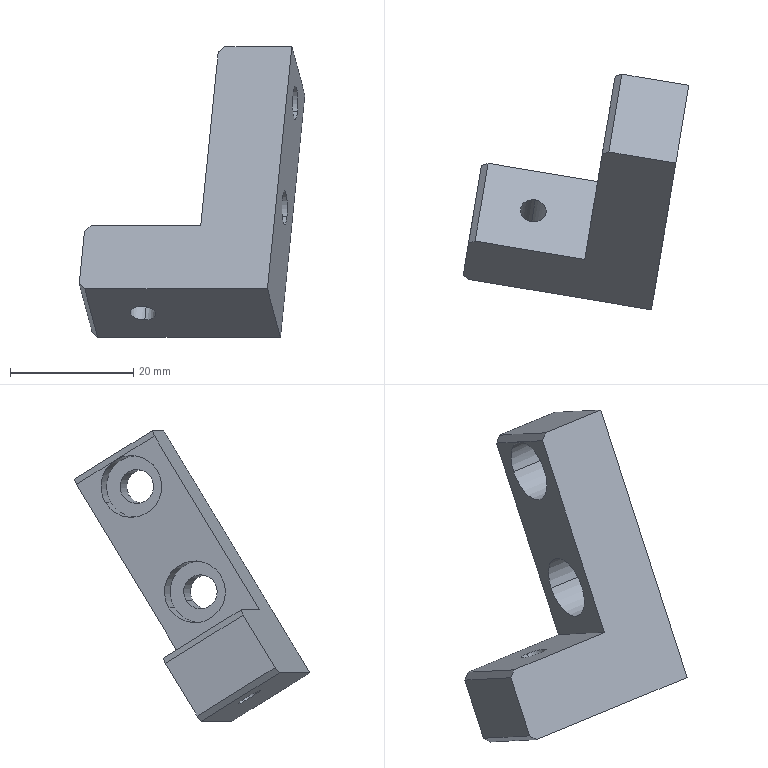Component | SolidWorks | 14AC-24-1-010-1 | 1 solid | 23 faces | box 36.54 x 38.12 x 47.06 mm | volume 10349 mm3 | plane 13 | cylinder 10 | commonest cylinder face diameters 10 x4 5.5 x4 4.2 x2
STEP:
#1=COLOUR_RGB('',0.7922,0.8196,0.9333);
#2=FILL_AREA_STYLE_COLOUR('',#1);
#3=FILL_AREA_STYLE('',(#2));
#4=SURFACE_STYLE_FILL_AREA(#3);
#5=SURFACE_SIDE_STYLE('',(#4));
#6=SURFACE_STYLE_USAGE(.BOTH.,#5);
#7=PRESENTATION_STYLE_ASSIGNMENT((#6));
#8=CARTESIAN_POINT('',(13.586,-5.303,-6.958));
#9=VERTEX_POINT('',#8);
#10=CARTESIAN_POINT('',(13.531,-5.634,-6.753));
#11=VERTEX_POINT('',#10);
#12=CARTESIAN_POINT('',(13.559,-5.468,-6.856));
#13=DIRECTION('',(-0.9864,0.1642,0.));
#14=DIRECTION('',(-0.1401,-0.8413,0.5222));
#15=AXIS2_PLACEMENT_3D('',#12,#13,#14);
#16=CIRCLE('',#15,0.1969);
#17=EDGE_CURVE('',#9,#11,#16,.T.);
#18=ORIENTED_EDGE('',*,*,#17,.F.);
#19=CARTESIAN_POINT('',(13.377,-5.268,-6.958));
#20=VERTEX_POINT('',#19);
#21=CARTESIAN_POINT('',(13.377,-5.268,-6.958));
#22=DIRECTION('',(-0.9864,0.1642,0.));
#23=VECTOR('',#22,39.37);
#24=LINE('',#21,#23);
#25=EDGE_CURVE('',#9,#20,#24,.T.);
#26=ORIENTED_EDGE('',*,*,#25,.T.);
#27=CARTESIAN_POINT('',(13.321,-5.599,-6.753));
#28=VERTEX_POINT('',#27);
#29=CARTESIAN_POINT('',(13.349,-5.433,-6.856));
#30=DIRECTION('',(-0.9864,0.1642,0.));
#31=DIRECTION('',(-0.1401,-0.8413,0.5222));
#32=AXIS2_PLACEMENT_3D('',#29,#30,#31);
#33=CIRCLE('',#32,0.1969);
#34=EDGE_CURVE('',#20,#28,#33,.T.);
#35=ORIENTED_EDGE('',*,*,#34,.T.);
#36=CARTESIAN_POINT('',(13.321,-5.599,-6.753));
#37=DIRECTION('',(-0.9864,0.1642,0.));
#38=VECTOR('',#37,39.37);
#39=LINE('',#36,#38);
#40=EDGE_CURVE('',#11,#28,#39,.T.);
#41=ORIENTED_EDGE('',*,*,#40,.F.);
#42=EDGE_LOOP('',(#18,#26,#35,#41));
#43=FACE_OUTER_BOUND('',#42,.T.);
#44=CARTESIAN_POINT('',(13.349,-5.433,-6.856));
#45=DIRECTION('',(-0.9864,0.1642,0.));
#46=DIRECTION('',(-0.1401,-0.8413,0.5222));
#47=AXIS2_PLACEMENT_3D('',#44,#45,#46);
#48=CYLINDRICAL_SURFACE('',#47,0.1969);
#49=ADVANCED_FACE('',(#43),#48,.F.);
#50=CARTESIAN_POINT('',(13.83,-5.42,-6.912));
#51=VERTEX_POINT('',#50);
#52=CARTESIAN_POINT('',(13.8,-5.602,-6.799));
#53=VERTEX_POINT('',#52);
#54=CARTESIAN_POINT('',(13.815,-5.511,-6.856));
#55=DIRECTION('',(-0.9864,0.1642,0.));
#56=DIRECTION('',(-0.1401,-0.8413,0.5222));
#57=AXIS2_PLACEMENT_3D('',#54,#55,#56);
#58=CIRCLE('',#57,0.1083);
#59=EDGE_CURVE('',#51,#53,#58,.T.);
#60=ORIENTED_EDGE('',*,*,#59,.F.);
#61=CARTESIAN_POINT('',(13.574,-5.377,-6.912));
#62=VERTEX_POINT('',#61);
#63=CARTESIAN_POINT('',(13.364,-5.342,-6.912));
#64=DIRECTION('',(-0.9864,0.1642,0.));
#65=VECTOR('',#64,39.37);
#66=LINE('',#63,#65);
#67=EDGE_CURVE('',#51,#62,#66,.T.);
#68=ORIENTED_EDGE('',*,*,#67,.T.);
#69=CARTESIAN_POINT('',(13.544,-5.559,-6.799));
#70=VERTEX_POINT('',#69);
#71=CARTESIAN_POINT('',(13.559,-5.468,-6.856));
#72=DIRECTION('',(-0.9864,0.1642,0.));
#73=DIRECTION('',(-0.1401,-0.8413,0.5222));
#74=AXIS2_PLACEMENT_3D('',#71,#72,#73);
#75=CIRCLE('',#74,0.1083);
#76=EDGE_CURVE('',#62,#70,#75,.T.);
#77=ORIENTED_EDGE('',*,*,#76,.T.);
#78=CARTESIAN_POINT('',(13.334,-5.525,-6.799));
#79=DIRECTION('',(-0.9864,0.1642,0.));
#80=VECTOR('',#79,39.37);
#81=LINE('',#78,#80);
#82=EDGE_CURVE('',#53,#70,#81,.T.);
#83=ORIENTED_EDGE('',*,*,#82,.F.);
#84=EDGE_LOOP('',(#60,#68,#77,#83));
#85=FACE_OUTER_BOUND('',#84,.T.);
#86=CARTESIAN_POINT('',(13.349,-5.433,-6.856));
#87=DIRECTION('',(-0.9864,0.1642,0.));
#88=DIRECTION('',(-0.1401,-0.8413,0.5222));
#89=AXIS2_PLACEMENT_3D('',#86,#87,#88);
#90=CYLINDRICAL_SURFACE('',#89,0.1083);
#91=ADVANCED_FACE('',(#85),#90,.F.);
#92=CARTESIAN_POINT('',(13.654,-4.897,-6.287));
#93=VERTEX_POINT('',#92);
#94=CARTESIAN_POINT('',(13.599,-5.228,-6.081));
#95=VERTEX_POINT('',#94);
#96=CARTESIAN_POINT('',(13.626,-5.063,-6.184));
#97=DIRECTION('',(-0.9864,0.1642,0.));
#98=DIRECTION('',(-0.1401,-0.8413,0.5222));
#99=AXIS2_PLACEMENT_3D('',#96,#97,#98);
#100=CIRCLE('',#99,0.1969);
#101=EDGE_CURVE('',#93,#95,#100,.T.);
#102=ORIENTED_EDGE('',*,*,#101,.F.);
#103=CARTESIAN_POINT('',(13.444,-4.862,-6.287));
#104=VERTEX_POINT('',#103);
#105=CARTESIAN_POINT('',(13.444,-4.862,-6.287));
#106=DIRECTION('',(-0.9864,0.1642,0.));
#107=VECTOR('',#106,39.37);
#108=LINE('',#105,#107);
#109=EDGE_CURVE('',#93,#104,#108,.T.);
#110=ORIENTED_EDGE('',*,*,#109,.T.);
#111=CARTESIAN_POINT('',(13.389,-5.194,-6.081));
#112=VERTEX_POINT('',#111);
#113=CARTESIAN_POINT('',(13.417,-5.028,-6.184));
#114=DIRECTION('',(-0.9864,0.1642,0.));
#115=DIRECTION('',(-0.1401,-0.8413,0.5222));
#116=AXIS2_PLACEMENT_3D('',#113,#114,#115);
#117=CIRCLE('',#116,0.1969);
#118=EDGE_CURVE('',#104,#112,#117,.T.);
#119=ORIENTED_EDGE('',*,*,#118,.T.);
#120=CARTESIAN_POINT('',(13.389,-5.194,-6.081));
#121=DIRECTION('',(-0.9864,0.1642,0.));
#122=VECTOR('',#121,39.37);
#123=LINE('',#120,#122);
#124=EDGE_CURVE('',#95,#112,#123,.T.);
#125=ORIENTED_EDGE('',*,*,#124,.F.);
#126=EDGE_LOOP('',(#102,#110,#119,#125));
#127=FACE_OUTER_BOUND('',#126,.T.);
#128=CARTESIAN_POINT('',(13.417,-5.028,-6.184));
#129=DIRECTION('',(-0.9864,0.1642,0.));
#130=DIRECTION('',(-0.1401,-0.8413,0.5222));
#131=AXIS2_PLACEMENT_3D('',#128,#129,#130);
#132=CYLINDRICAL_SURFACE('',#131,0.1969);
#133=ADVANCED_FACE('',(#127),#132,.F.);
#134=CARTESIAN_POINT('',(13.898,-5.014,-6.241));
#135=VERTEX_POINT('',#134);
#136=CARTESIAN_POINT('',(13.867,-5.197,-6.127));
#137=VERTEX_POINT('',#136);
#138=CARTESIAN_POINT('',(13.883,-5.106,-6.184));
#139=DIRECTION('',(-0.9864,0.1642,0.));
#140=DIRECTION('',(-0.1401,-0.8413,0.5222));
#141=AXIS2_PLACEMENT_3D('',#138,#139,#140);
#142=CIRCLE('',#141,0.1083);
#143=EDGE_CURVE('',#135,#137,#142,.T.);
#144=ORIENTED_EDGE('',*,*,#143,.F.);
#145=CARTESIAN_POINT('',(13.641,-4.972,-6.241));
#146=VERTEX_POINT('',#145);
#147=CARTESIAN_POINT('',(13.432,-4.937,-6.241));
#148=DIRECTION('',(-0.9864,0.1642,0.));
#149=VECTOR('',#148,39.37);
#150=LINE('',#147,#149);
#151=EDGE_CURVE('',#135,#146,#150,.T.);
#152=ORIENTED_EDGE('',*,*,#151,.T.);
#153=CARTESIAN_POINT('',(13.611,-5.154,-6.127));
#154=VERTEX_POINT('',#153);
#155=CARTESIAN_POINT('',(13.626,-5.063,-6.184));
#156=DIRECTION('',(-0.9864,0.1642,0.));
#157=DIRECTION('',(-0.1401,-0.8413,0.5222));
#158=AXIS2_PLACEMENT_3D('',#155,#156,#157);
#159=CIRCLE('',#158,0.1083);
#160=EDGE_CURVE('',#146,#154,#159,.T.);
#161=ORIENTED_EDGE('',*,*,#160,.T.);
#162=CARTESIAN_POINT('',(13.401,-5.119,-6.127));
#163=DIRECTION('',(-0.9864,0.1642,0.));
#164=VECTOR('',#163,39.37);
#165=LINE('',#162,#164);
#166=EDGE_CURVE('',#137,#154,#165,.T.);
#167=ORIENTED_EDGE('',*,*,#166,.F.);
#168=EDGE_LOOP('',(#144,#152,#161,#167));
#169=FACE_OUTER_BOUND('',#168,.T.);
#170=CARTESIAN_POINT('',(13.417,-5.028,-6.184));
#171=DIRECTION('',(-0.9864,0.1642,0.));
#172=DIRECTION('',(-0.1401,-0.8413,0.5222));
#173=AXIS2_PLACEMENT_3D('',#170,#171,#172);
#174=CYLINDRICAL_SURFACE('',#173,0.1083);
#175=ADVANCED_FACE('',(#169),#174,.F.);
#176=CARTESIAN_POINT('',(12.924,-5.708,-7.57));
#177=VERTEX_POINT('',#176);
#178=CARTESIAN_POINT('',(12.901,-5.847,-7.484));
#179=VERTEX_POINT('',#178);
#180=CARTESIAN_POINT('',(12.913,-5.778,-7.527));
#181=DIRECTION('',(0.08576,0.5151,0.8529));
#182=DIRECTION('',(0.9864,-0.1642,0.));
#183=AXIS2_PLACEMENT_3D('',#180,#181,#182);
#184=CIRCLE('',#183,0.08268);
#185=EDGE_CURVE('',#177,#179,#184,.T.);
#186=ORIENTED_EDGE('',*,*,#185,.F.);
#187=CARTESIAN_POINT('',(12.965,-5.465,-7.167));
#188=VERTEX_POINT('',#187);
#189=CARTESIAN_POINT('',(12.965,-5.465,-7.167));
#190=DIRECTION('',(0.08576,0.5151,0.8529));
#191=VECTOR('',#190,39.37);
#192=LINE('',#189,#191);
#193=EDGE_CURVE('',#177,#188,#192,.T.);
#194=ORIENTED_EDGE('',*,*,#193,.T.);
#195=CARTESIAN_POINT('',(12.941,-5.604,-7.081));
#196=VERTEX_POINT('',#195);
#197=CARTESIAN_POINT('',(12.953,-5.534,-7.124));
#198=DIRECTION('',(0.08576,0.5151,0.8529));
#199=DIRECTION('',(-0.1401,-0.8413,0.5222));
#200=AXIS2_PLACEMENT_3D('',#197,#198,#199);
#201=CIRCLE('',#200,0.08268);
#202=EDGE_CURVE('',#188,#196,#201,.T.);
#203=ORIENTED_EDGE('',*,*,#202,.T.);
#204=CARTESIAN_POINT('',(12.941,-5.604,-7.081));
#205=DIRECTION('',(0.08576,0.5151,0.8529));
#206=VECTOR('',#205,39.37);
#207=LINE('',#204,#206);
#208=EDGE_CURVE('',#179,#196,#207,.T.);
#209=ORIENTED_EDGE('',*,*,#208,.F.);
#210=EDGE_LOOP('',(#186,#194,#203,#209));
#211=FACE_OUTER_BOUND('',#210,.T.);
#212=CARTESIAN_POINT('',(12.953,-5.534,-7.124));
#213=DIRECTION('',(0.08576,0.5151,0.8529));
#214=DIRECTION('',(-0.1401,-0.8413,0.5222));
#215=AXIS2_PLACEMENT_3D('',#212,#213,#214);
#216=CYLINDRICAL_SURFACE('',#215,0.08268);
#217=ADVANCED_FACE('',(#211),#216,.F.);
#218=CARTESIAN_POINT('',(13.517,-4.664,-6.137));
#219=VERTEX_POINT('',#218);
#220=CARTESIAN_POINT('',(13.944,-4.735,-6.137));
#221=VERTEX_POINT('',#220);
#222=CARTESIAN_POINT('',(13.944,-4.735,-6.137));
#223=DIRECTION('',(0.9864,-0.1642,-0.));
#224=VECTOR('',#223,39.37);
#225=LINE('',#222,#224);
#226=EDGE_CURVE('',#219,#221,#225,.T.);
#227=ORIENTED_EDGE('',*,*,#226,.F.);
#228=CARTESIAN_POINT('',(13.434,-5.161,-5.828));
#229=VERTEX_POINT('',#228);
#230=CARTESIAN_POINT('',(13.517,-4.664,-6.137));
#231=DIRECTION('',(-0.1401,-0.8413,0.5222));
#232=VECTOR('',#231,39.37);
#233=LINE('',#230,#232);
#234=EDGE_CURVE('',#219,#229,#233,.T.);
#235=ORIENTED_EDGE('',*,*,#234,.T.);
#236=CARTESIAN_POINT('',(13.861,-5.232,-5.828));
#237=VERTEX_POINT('',#236);
#238=CARTESIAN_POINT('',(13.861,-5.232,-5.828));
#239=DIRECTION('',(0.9864,-0.1642,-0.));
#240=VECTOR('',#239,39.37);
#241=LINE('',#238,#240);
#242=EDGE_CURVE('',#229,#237,#241,.T.);
#243=ORIENTED_EDGE('',*,*,#242,.T.);
#244=CARTESIAN_POINT('',(13.944,-4.735,-6.137));
#245=DIRECTION('',(-0.1401,-0.8413,0.5222));
#246=VECTOR('',#245,39.37);
#247=LINE('',#244,#246);
#248=EDGE_CURVE('',#221,#237,#247,.T.);
#249=ORIENTED_EDGE('',*,*,#248,.F.);
#250=EDGE_LOOP('',(#227,#235,#243,#249));
#251=FACE_OUTER_BOUND('',#250,.T.);
#252=CARTESIAN_POINT('',(13.944,-4.735,-6.137));
#253=DIRECTION('',(-0.08576,-0.5151,-0.8529));
#254=DIRECTION('',(-0.9864,0.1642,0.));
#255=AXIS2_PLACEMENT_3D('',#252,#253,#254);
#256=PLANE('',#255);
#257=ADVANCED_FACE('',(#251),#256,.F.);
#258=CARTESIAN_POINT('',(13.815,-5.511,-6.856));
#259=DIRECTION('',(-0.9864,0.1642,0.));
#260=DIRECTION('',(-0.1401,-0.8413,0.5222));
#261=AXIS2_PLACEMENT_3D('',#258,#259,#260);
#262=CIRCLE('',#261,0.1083);
#263=EDGE_CURVE('',#53,#51,#262,.T.);
#264=ORIENTED_EDGE('',*,*,#263,.T.);
#265=ORIENTED_EDGE('',*,*,#59,.T.);
#266=EDGE_LOOP('',(#264,#265));
#267=FACE_BOUND('',#266,.T.);
#268=CARTESIAN_POINT('',(13.883,-5.106,-6.184));
#269=DIRECTION('',(-0.9864,0.1642,0.));
#270=DIRECTION('',(-0.1401,-0.8413,0.5222));
#271=AXIS2_PLACEMENT_3D('',#268,#269,#270);
#272=CIRCLE('',#271,0.1083);
#273=EDGE_CURVE('',#137,#135,#272,.T.);
#274=ORIENTED_EDGE('',*,*,#273,.T.);
#275=ORIENTED_EDGE('',*,*,#143,.T.);
#276=EDGE_LOOP('',(#274,#275));
#277=FACE_BOUND('',#276,.T.);
#278=CARTESIAN_POINT('',(13.706,-6.165,-7.373));
#279=VERTEX_POINT('',#278);
#280=CARTESIAN_POINT('',(13.706,-6.165,-7.373));
#281=DIRECTION('',(-0.08576,-0.5151,-0.8529));
#282=VECTOR('',#281,39.37);
#283=LINE('',#280,#282);
#284=EDGE_CURVE('',#237,#279,#283,.T.);
#285=ORIENTED_EDGE('',*,*,#284,.T.);
#286=CARTESIAN_POINT('',(13.789,-5.668,-7.681));
#287=VERTEX_POINT('',#286);
#288=CARTESIAN_POINT('',(13.789,-5.668,-7.681));
#289=DIRECTION('',(-0.1401,-0.8413,0.5222));
#290=VECTOR('',#289,39.37);
#291=LINE('',#288,#290);
#292=EDGE_CURVE('',#287,#279,#291,.T.);
#293=ORIENTED_EDGE('',*,*,#292,.F.);
#294=CARTESIAN_POINT('',(13.789,-5.668,-7.681));
#295=DIRECTION('',(-0.08576,-0.5151,-0.8529));
#296=VECTOR('',#295,39.37);
#297=LINE('',#294,#296);
#298=EDGE_CURVE('',#221,#287,#297,.T.);
#299=ORIENTED_EDGE('',*,*,#298,.F.);
#300=ORIENTED_EDGE('',*,*,#248,.T.);
#301=EDGE_LOOP('',(#285,#293,#299,#300));
#302=FACE_OUTER_BOUND('',#301,.T.);
#303=CARTESIAN_POINT('',(13.789,-5.668,-7.681));
#304=DIRECTION('',(-0.9864,0.1642,0.));
#305=DIRECTION('',(-0.1401,-0.8413,0.5222));
#306=AXIS2_PLACEMENT_3D('',#303,#304,#305);
#307=PLANE('',#306);
#308=ADVANCED_FACE('',(#267,#277,#302),#307,.F.);
#309=CARTESIAN_POINT('',(12.913,-5.778,-7.527));
#310=DIRECTION('',(0.08576,0.5151,0.8529));
#311=DIRECTION('',(0.9864,-0.1642,0.));
#312=AXIS2_PLACEMENT_3D('',#309,#310,#311);
#313=CIRCLE('',#312,0.08268);
#314=EDGE_CURVE('',#179,#177,#313,.T.);
#315=ORIENTED_EDGE('',*,*,#314,.T.);
#316=ORIENTED_EDGE('',*,*,#185,.T.);
#317=EDGE_LOOP('',(#315,#316));
#318=FACE_BOUND('',#317,.T.);
#319=CARTESIAN_POINT('',(12.541,-5.971,-7.373));
#320=VERTEX_POINT('',#319);
#321=CARTESIAN_POINT('',(13.706,-6.165,-7.373));
#322=DIRECTION('',(-0.9864,0.1642,0.));
#323=VECTOR('',#322,39.37);
#324=LINE('',#321,#323);
#325=EDGE_CURVE('',#279,#320,#324,.T.);
#326=ORIENTED_EDGE('',*,*,#325,.T.);
#327=CARTESIAN_POINT('',(12.624,-5.474,-7.681));
#328=VERTEX_POINT('',#327);
#329=CARTESIAN_POINT('',(12.624,-5.474,-7.681));
#330=DIRECTION('',(0.1401,0.8413,-0.5222));
#331=VECTOR('',#330,39.37);
#332=LINE('',#329,#331);
#333=EDGE_CURVE('',#320,#328,#332,.T.);
#334=ORIENTED_EDGE('',*,*,#333,.T.);
#335=CARTESIAN_POINT('',(13.789,-5.668,-7.681));
#336=DIRECTION('',(-0.9864,0.1642,0.));
#337=VECTOR('',#336,39.37);
#338=LINE('',#335,#337);
#339=EDGE_CURVE('',#287,#328,#338,.T.);
#340=ORIENTED_EDGE('',*,*,#339,.F.);
#341=ORIENTED_EDGE('',*,*,#292,.T.);
#342=EDGE_LOOP('',(#326,#334,#340,#341));
#343=FACE_OUTER_BOUND('',#342,.T.);
#344=CARTESIAN_POINT('',(13.789,-5.668,-7.681));
#345=DIRECTION('',(0.08576,0.5151,0.8529));
#346=DIRECTION('',(0.9864,-0.1642,-0.));
#347=AXIS2_PLACEMENT_3D('',#344,#345,#346);
#348=PLANE('',#347);
#349=ADVANCED_FACE('',(#318,#343),#348,.F.);
#350=CARTESIAN_POINT('',(12.588,-5.447,-7.648));
#351=VERTEX_POINT('',#350);
#352=CARTESIAN_POINT('',(12.622,-5.245,-7.312));
#353=VERTEX_POINT('',#352);
#354=CARTESIAN_POINT('',(12.585,-5.468,-7.681));
#355=DIRECTION('',(0.08576,0.5151,0.8529));
#356=VECTOR('',#355,39.37);
#357=LINE('',#354,#356);
#358=EDGE_CURVE('',#351,#353,#357,.T.);
#359=ORIENTED_EDGE('',*,*,#358,.F.);
#360=CARTESIAN_POINT('',(12.506,-5.944,-7.339));
#361=VERTEX_POINT('',#360);
#362=CARTESIAN_POINT('',(12.588,-5.447,-7.648));
#363=DIRECTION('',(-0.1401,-0.8413,0.5222));
#364=VECTOR('',#363,39.37);
#365=LINE('',#362,#364);
#366=EDGE_CURVE('',#351,#361,#365,.T.);
#367=ORIENTED_EDGE('',*,*,#366,.T.);
#368=CARTESIAN_POINT('',(12.539,-5.742,-7.004));
#369=VERTEX_POINT('',#368);
#370=CARTESIAN_POINT('',(12.502,-5.965,-7.373));
#371=DIRECTION('',(0.08576,0.5151,0.8529));
#372=VECTOR('',#371,39.37);
#373=LINE('',#370,#372);
#374=EDGE_CURVE('',#361,#369,#373,.T.);
#375=ORIENTED_EDGE('',*,*,#374,.T.);
#376=CARTESIAN_POINT('',(12.622,-5.245,-7.312));
#377=DIRECTION('',(0.1401,0.8413,-0.5222));
#378=VECTOR('',#377,39.37);
#379=LINE('',#376,#378);
#380=EDGE_CURVE('',#369,#353,#379,.T.);
#381=ORIENTED_EDGE('',*,*,#380,.T.);
#382=EDGE_LOOP('',(#359,#367,#375,#381));
#383=FACE_OUTER_BOUND('',#382,.T.);
#384=CARTESIAN_POINT('',(12.585,-5.468,-7.681));
#385=DIRECTION('',(0.9864,-0.1642,-0.));
#386=DIRECTION('',(0.1401,0.8413,-0.5222));
#387=AXIS2_PLACEMENT_3D('',#384,#385,#386);
#388=PLANE('',#387);
#389=ADVANCED_FACE('',(#383),#388,.F.);
#390=ORIENTED_EDGE('',*,*,#339,.T.);
#391=CARTESIAN_POINT('',(12.473,-5.361,-7.539));
#392=DIRECTION('',(-0.6369,0.4803,0.6031));
#393=VECTOR('',#392,39.37);
#394=LINE('',#391,#393);
#395=EDGE_CURVE('',#328,#351,#394,.T.);
#396=ORIENTED_EDGE('',*,*,#395,.T.);
#397=ORIENTED_EDGE('',*,*,#358,.T.);
#398=CARTESIAN_POINT('',(12.664,-5.231,-7.278));
#399=VERTEX_POINT('',#398);
#400=CARTESIAN_POINT('',(13.203,-5.055,-6.85));
#401=DIRECTION('',(0.7581,0.2481,0.6031));
#402=VECTOR('',#401,39.37);
#403=LINE('',#400,#402);
#404=EDGE_CURVE('',#353,#399,#403,.T.);
#405=ORIENTED_EDGE('',*,*,#404,.T.);
#406=CARTESIAN_POINT('',(13.363,-5.347,-7.278));
#407=VERTEX_POINT('',#406);
#408=CARTESIAN_POINT('',(13.363,-5.347,-7.278));
#409=DIRECTION('',(-0.9864,0.1642,0.));
#410=VECTOR('',#409,39.37);
#411=LINE('',#408,#410);
#412=EDGE_CURVE('',#407,#399,#411,.T.);
#413=ORIENTED_EDGE('',*,*,#412,.F.);
#414=CARTESIAN_POINT('',(13.475,-4.678,-6.17));
#415=VERTEX_POINT('',#414);
#416=CARTESIAN_POINT('',(13.478,-4.658,-6.137));
#417=DIRECTION('',(-0.08576,-0.5151,-0.8529));
#418=VECTOR('',#417,39.37);
#419=LINE('',#416,#418);
#420=EDGE_CURVE('',#415,#407,#419,.T.);
#421=ORIENTED_EDGE('',*,*,#420,.F.);
#422=CARTESIAN_POINT('',(12.937,-4.854,-6.598));
#423=DIRECTION('',(0.7581,0.2481,0.6031));
#424=VECTOR('',#423,39.37);
#425=LINE('',#422,#424);
#426=EDGE_CURVE('',#415,#219,#425,.T.);
#427=ORIENTED_EDGE('',*,*,#426,.T.);
#428=ORIENTED_EDGE('',*,*,#226,.T.);
#429=ORIENTED_EDGE('',*,*,#298,.T.);
#430=EDGE_LOOP('',(#390,#396,#397,#405,#413,#421,#427,#428,#429));
#431=FACE_OUTER_BOUND('',#430,.T.);
#432=CARTESIAN_POINT('',(13.265,-5.102,-6.909));
#433=DIRECTION('',(0.1401,0.8413,-0.5222));
#434=DIRECTION('',(0.08576,0.5151,0.8529));
#435=AXIS2_PLACEMENT_3D('',#432,#433,#434);
#436=PLANE('',#435);
#437=ADVANCED_FACE('',(#431),#436,.T.);
#438=ORIENTED_EDGE('',*,*,#374,.F.);
#439=CARTESIAN_POINT('',(12.506,-5.944,-7.339));
#440=DIRECTION('',(0.6369,-0.4803,-0.6031));
#441=VECTOR('',#440,39.37);
#442=LINE('',#439,#441);
#443=EDGE_CURVE('',#361,#320,#442,.T.);
#444=ORIENTED_EDGE('',*,*,#443,.T.);
#445=ORIENTED_EDGE('',*,*,#325,.F.);
#446=ORIENTED_EDGE('',*,*,#284,.F.);
#447=ORIENTED_EDGE('',*,*,#242,.F.);
#448=CARTESIAN_POINT('',(13.392,-5.175,-5.862));
#449=VERTEX_POINT('',#448);
#450=CARTESIAN_POINT('',(13.392,-5.175,-5.862));
#451=DIRECTION('',(-0.7581,-0.2481,-0.6031));
#452=VECTOR('',#451,39.37);
#453=LINE('',#450,#452);
#454=EDGE_CURVE('',#229,#449,#453,.T.);
#455=ORIENTED_EDGE('',*,*,#454,.T.);
#456=CARTESIAN_POINT('',(13.281,-5.844,-6.97));
#457=VERTEX_POINT('',#456);
#458=CARTESIAN_POINT('',(13.395,-5.155,-5.828));
#459=DIRECTION('',(0.08576,0.5151,0.8529));
#460=VECTOR('',#459,39.37);
#461=LINE('',#458,#460);
#462=EDGE_CURVE('',#457,#449,#461,.T.);
#463=ORIENTED_EDGE('',*,*,#462,.F.);
#464=CARTESIAN_POINT('',(12.582,-5.728,-6.97));
#465=VERTEX_POINT('',#464);
#466=CARTESIAN_POINT('',(13.281,-5.844,-6.97));
#467=DIRECTION('',(-0.9864,0.1642,0.));
#468=VECTOR('',#467,39.37);
#469=LINE('',#466,#468);
#470=EDGE_CURVE('',#457,#465,#469,.T.);
#471=ORIENTED_EDGE('',*,*,#470,.T.);
#472=CARTESIAN_POINT('',(12.582,-5.728,-6.97));
#473=DIRECTION('',(-0.7581,-0.2481,-0.6031));
#474=VECTOR('',#473,39.37);
#475=LINE('',#472,#474);
#476=EDGE_CURVE('',#465,#369,#475,.T.);
#477=ORIENTED_EDGE('',*,*,#476,.T.);
#478=EDGE_LOOP('',(#438,#444,#445,#446,#447,#455,#463,#471,#477));
#479=FACE_OUTER_BOUND('',#478,.T.);
#480=CARTESIAN_POINT('',(13.182,-5.598,-6.601));
#481=DIRECTION('',(0.1401,0.8413,-0.5222));
#482=DIRECTION('',(0.08576,0.5151,0.8529));
#483=AXIS2_PLACEMENT_3D('',#480,#481,#482);
#484=PLANE('',#483);
#485=ADVANCED_FACE('',(#479),#484,.F.);
#486=CARTESIAN_POINT('',(12.953,-5.534,-7.124));
#487=DIRECTION('',(0.08576,0.5151,0.8529));
#488=DIRECTION('',(-0.1401,-0.8413,0.5222));
#489=AXIS2_PLACEMENT_3D('',#486,#487,#488);
#490=CIRCLE('',#489,0.08268);
#491=EDGE_CURVE('',#196,#188,#490,.T.);
#492=ORIENTED_EDGE('',*,*,#491,.F.);
#493=ORIENTED_EDGE('',*,*,#202,.F.);
#494=EDGE_LOOP('',(#492,#493));
#495=FACE_BOUND('',#494,.T.);
#496=ORIENTED_EDGE('',*,*,#412,.T.);
#497=CARTESIAN_POINT('',(12.664,-5.231,-7.278));
#498=DIRECTION('',(-0.1401,-0.8413,0.5222));
#499=VECTOR('',#498,39.37);
#500=LINE('',#497,#499);
#501=EDGE_CURVE('',#399,#465,#500,.T.);
#502=ORIENTED_EDGE('',*,*,#501,.T.);
#503=ORIENTED_EDGE('',*,*,#470,.F.);
#504=CARTESIAN_POINT('',(13.363,-5.347,-7.278));
#505=DIRECTION('',(-0.1401,-0.8413,0.5222));
#506=VECTOR('',#505,39.37);
#507=LINE('',#504,#506);
#508=EDGE_CURVE('',#407,#457,#507,.T.);
#509=ORIENTED_EDGE('',*,*,#508,.F.);
#510=EDGE_LOOP('',(#496,#502,#503,#509));
#511=FACE_OUTER_BOUND('',#510,.T.);
#512=CARTESIAN_POINT('',(13.363,-5.347,-7.278));
#513=DIRECTION('',(-0.08576,-0.5151,-0.8529));
#514=DIRECTION('',(0.1401,0.8413,-0.5222));
#515=AXIS2_PLACEMENT_3D('',#512,#513,#514);
#516=PLANE('',#515);
#517=ADVANCED_FACE('',(#495,#511),#516,.F.);
#518=CARTESIAN_POINT('',(13.349,-5.433,-6.856));
#519=DIRECTION('',(-0.9864,0.1642,0.));
#520=DIRECTION('',(-0.1401,-0.8413,0.5222));
#521=AXIS2_PLACEMENT_3D('',#518,#519,#520);
#522=CIRCLE('',#521,0.1969);
#523=EDGE_CURVE('',#28,#20,#522,.T.);
#524=ORIENTED_EDGE('',*,*,#523,.F.);
#525=ORIENTED_EDGE('',*,*,#34,.F.);
#526=EDGE_LOOP('',(#524,#525));
#527=FACE_BOUND('',#526,.T.);
#528=ORIENTED_EDGE('',*,*,#462,.T.);
#529=CARTESIAN_POINT('',(13.433,-4.927,-6.016));
#530=VERTEX_POINT('',#529);
#531=CARTESIAN_POINT('',(13.392,-5.175,-5.862));
#532=DIRECTION('',(0.1401,0.8413,-0.5222));
#533=VECTOR('',#532,39.37);
#534=LINE('',#531,#533);
#535=EDGE_CURVE('',#449,#530,#534,.T.);
#536=ORIENTED_EDGE('',*,*,#535,.T.);
#537=CARTESIAN_POINT('',(13.417,-5.028,-6.184));
#538=DIRECTION('',(-0.9864,0.1642,0.));
#539=DIRECTION('',(-0.1401,-0.8413,0.5222));
#540=AXIS2_PLACEMENT_3D('',#537,#538,#539);
#541=CIRCLE('',#540,0.1969);
#542=EDGE_CURVE('',#112,#530,#541,.T.);
#543=ORIENTED_EDGE('',*,*,#542,.F.);
#544=ORIENTED_EDGE('',*,*,#118,.F.);
#545=CARTESIAN_POINT('',(13.417,-5.028,-6.184));
#546=DIRECTION('',(-0.9864,0.1642,0.));
#547=DIRECTION('',(-0.1401,-0.8413,0.5222));
#548=AXIS2_PLACEMENT_3D('',#545,#546,#547);
#549=CIRCLE('',#548,0.1969);
#550=EDGE_CURVE('',#530,#104,#549,.T.);
#551=ORIENTED_EDGE('',*,*,#550,.F.);
#552=CARTESIAN_POINT('',(13.392,-5.175,-5.862));
#553=DIRECTION('',(0.1401,0.8413,-0.5222));
#554=VECTOR('',#553,39.37);
#555=LINE('',#552,#554);
#556=EDGE_CURVE('',#530,#415,#555,.T.);
#557=ORIENTED_EDGE('',*,*,#556,.T.);
#558=ORIENTED_EDGE('',*,*,#420,.T.);
#559=ORIENTED_EDGE('',*,*,#508,.T.);
#560=EDGE_LOOP('',(#528,#536,#543,#544,#551,#557,#558,#559));
#561=FACE_OUTER_BOUND('',#560,.T.);
#562=CARTESIAN_POINT('',(13.318,-5.621,-6.601));
#563=DIRECTION('',(0.9864,-0.1642,-0.));
#564=DIRECTION('',(0.1401,0.8413,-0.5222));
#565=AXIS2_PLACEMENT_3D('',#562,#563,#564);
#566=PLANE('',#565);
#567=ADVANCED_FACE('',(#527,#561),#566,.F.);
#568=ORIENTED_EDGE('',*,*,#193,.F.);
#569=ORIENTED_EDGE('',*,*,#314,.F.);
#570=ORIENTED_EDGE('',*,*,#208,.T.);
#571=ORIENTED_EDGE('',*,*,#491,.T.);
#572=EDGE_LOOP('',(#568,#569,#570,#571));
#573=FACE_OUTER_BOUND('',#572,.T.);
#574=CARTESIAN_POINT('',(12.953,-5.534,-7.124));
#575=DIRECTION('',(0.08576,0.5151,0.8529));
#576=DIRECTION('',(-0.1401,-0.8413,0.5222));
#577=AXIS2_PLACEMENT_3D('',#574,#575,#576);
#578=CYLINDRICAL_SURFACE('',#577,0.08268);
#579=ADVANCED_FACE('',(#573),#578,.F.);
#580=ORIENTED_EDGE('',*,*,#151,.F.);
#581=ORIENTED_EDGE('',*,*,#273,.F.);
#582=ORIENTED_EDGE('',*,*,#166,.T.);
#583=CARTESIAN_POINT('',(13.626,-5.063,-6.184));
#584=DIRECTION('',(-0.9864,0.1642,0.));
#585=DIRECTION('',(-0.1401,-0.8413,0.5222));
#586=AXIS2_PLACEMENT_3D('',#583,#584,#585);
#587=CIRCLE('',#586,0.1083);
#588=EDGE_CURVE('',#154,#146,#587,.T.);
#589=ORIENTED_EDGE('',*,*,#588,.T.);
#590=EDGE_LOOP('',(#580,#581,#582,#589));
#591=FACE_OUTER_BOUND('',#590,.T.);
#592=CARTESIAN_POINT('',(13.417,-5.028,-6.184));
#593=DIRECTION('',(-0.9864,0.1642,0.));
#594=DIRECTION('',(-0.1401,-0.8413,0.5222));
#595=AXIS2_PLACEMENT_3D('',#592,#593,#594);
#596=CYLINDRICAL_SURFACE('',#595,0.1083);
#597=ADVANCED_FACE('',(#591),#596,.F.);
#598=ORIENTED_EDGE('',*,*,#588,.F.);
#599=ORIENTED_EDGE('',*,*,#160,.F.);
#600=EDGE_LOOP('',(#598,#599));
#601=FACE_BOUND('',#600,.T.);
#602=CARTESIAN_POINT('',(13.626,-5.063,-6.184));
#603=DIRECTION('',(-0.9864,0.1642,0.));
#604=DIRECTION('',(-0.1401,-0.8413,0.5222));
#605=AXIS2_PLACEMENT_3D('',#602,#603,#604);
#606=CIRCLE('',#605,0.1969);
#607=EDGE_CURVE('',#95,#93,#606,.T.);
#608=ORIENTED_EDGE('',*,*,#607,.T.);
#609=ORIENTED_EDGE('',*,*,#101,.T.);
#610=EDGE_LOOP('',(#608,#609));
#611=FACE_OUTER_BOUND('',#610,.T.);
#612=CARTESIAN_POINT('',(13.636,-5.007,-6.092));
#613=DIRECTION('',(0.9864,-0.1642,-0.));
#614=DIRECTION('',(0.1401,0.8413,-0.5222));
#615=AXIS2_PLACEMENT_3D('',#612,#613,#614);
#616=PLANE('',#615);
#617=ADVANCED_FACE('',(#601,#611),#616,.F.);
#618=ORIENTED_EDGE('',*,*,#109,.F.);
#619=ORIENTED_EDGE('',*,*,#607,.F.);
#620=ORIENTED_EDGE('',*,*,#124,.T.);
#621=ORIENTED_EDGE('',*,*,#542,.T.);
#622=ORIENTED_EDGE('',*,*,#550,.T.);
#623=EDGE_LOOP('',(#618,#619,#620,#621,#622));
#624=FACE_OUTER_BOUND('',#623,.T.);
#625=CARTESIAN_POINT('',(13.417,-5.028,-6.184));
#626=DIRECTION('',(-0.9864,0.1642,0.));
#627=DIRECTION('',(-0.1401,-0.8413,0.5222));
#628=AXIS2_PLACEMENT_3D('',#625,#626,#627);
#629=CYLINDRICAL_SURFACE('',#628,0.1969);
#630=ADVANCED_FACE('',(#624),#629,.F.);
#631=ORIENTED_EDGE('',*,*,#67,.F.);
#632=ORIENTED_EDGE('',*,*,#263,.F.);
#633=ORIENTED_EDGE('',*,*,#82,.T.);
#634=CARTESIAN_POINT('',(13.559,-5.468,-6.856));
#635=DIRECTION('',(-0.9864,0.1642,0.));
#636=DIRECTION('',(-0.1401,-0.8413,0.5222));
#637=AXIS2_PLACEMENT_3D('',#634,#635,#636);
#638=CIRCLE('',#637,0.1083);
#639=EDGE_CURVE('',#70,#62,#638,.T.);
#640=ORIENTED_EDGE('',*,*,#639,.T.);
#641=EDGE_LOOP('',(#631,#632,#633,#640));
#642=FACE_OUTER_BOUND('',#641,.T.);
#643=CARTESIAN_POINT('',(13.349,-5.433,-6.856));
#644=DIRECTION('',(-0.9864,0.1642,0.));
#645=DIRECTION('',(-0.1401,-0.8413,0.5222));
#646=AXIS2_PLACEMENT_3D('',#643,#644,#645);
#647=CYLINDRICAL_SURFACE('',#646,0.1083);
#648=ADVANCED_FACE('',(#642),#647,.F.);
#649=ORIENTED_EDGE('',*,*,#639,.F.);
#650=ORIENTED_EDGE('',*,*,#76,.F.);
#651=EDGE_LOOP('',(#649,#650));
#652=FACE_BOUND('',#651,.T.);
#653=CARTESIAN_POINT('',(13.559,-5.468,-6.856));
#654=DIRECTION('',(-0.9864,0.1642,0.));
#655=DIRECTION('',(-0.1401,-0.8413,0.5222));
#656=AXIS2_PLACEMENT_3D('',#653,#654,#655);
#657=CIRCLE('',#656,0.1969);
#658=EDGE_CURVE('',#11,#9,#657,.T.);
#659=ORIENTED_EDGE('',*,*,#658,.T.);
#660=ORIENTED_EDGE('',*,*,#17,.T.);
#661=EDGE_LOOP('',(#659,#660));
#662=FACE_OUTER_BOUND('',#661,.T.);
#663=CARTESIAN_POINT('',(13.568,-5.413,-6.763));
#664=DIRECTION('',(0.9864,-0.1642,-0.));
#665=DIRECTION('',(0.1401,0.8413,-0.5222));
#666=AXIS2_PLACEMENT_3D('',#663,#664,#665);
#667=PLANE('',#666);
#668=ADVANCED_FACE('',(#652,#662),#667,.F.);
#669=ORIENTED_EDGE('',*,*,#25,.F.);
#670=ORIENTED_EDGE('',*,*,#658,.F.);
#671=ORIENTED_EDGE('',*,*,#40,.T.);
#672=ORIENTED_EDGE('',*,*,#523,.T.);
#673=EDGE_LOOP('',(#669,#670,#671,#672));
#674=FACE_OUTER_BOUND('',#673,.T.);
#675=CARTESIAN_POINT('',(13.349,-5.433,-6.856));
#676=DIRECTION('',(-0.9864,0.1642,0.));
#677=DIRECTION('',(-0.1401,-0.8413,0.5222));
#678=AXIS2_PLACEMENT_3D('',#675,#676,#677);
#679=CYLINDRICAL_SURFACE('',#678,0.1969);
#680=ADVANCED_FACE('',(#674),#679,.F.);
#681=ORIENTED_EDGE('',*,*,#395,.F.);
#682=ORIENTED_EDGE('',*,*,#333,.F.);
#683=ORIENTED_EDGE('',*,*,#443,.F.);
#684=ORIENTED_EDGE('',*,*,#366,.F.);
#685=EDGE_LOOP('',(#681,#682,#683,#684));
#686=FACE_OUTER_BOUND('',#685,.T.);
#687=CARTESIAN_POINT('',(12.588,-5.447,-7.648));
#688=DIRECTION('',(0.7581,0.2481,0.6031));
#689=DIRECTION('',(-0.1401,-0.8413,0.5222));
#690=AXIS2_PLACEMENT_3D('',#687,#688,#689);
#691=PLANE('',#690);
#692=ADVANCED_FACE('',(#686),#691,.F.);
#693=ORIENTED_EDGE('',*,*,#404,.F.);
#694=ORIENTED_EDGE('',*,*,#380,.F.);
#695=ORIENTED_EDGE('',*,*,#476,.F.);
#696=ORIENTED_EDGE('',*,*,#501,.F.);
#697=EDGE_LOOP('',(#693,#694,#695,#696));
#698=FACE_OUTER_BOUND('',#697,.T.);
#699=CARTESIAN_POINT('',(12.664,-5.231,-7.278));
#700=DIRECTION('',(0.6369,-0.4803,-0.6031));
#701=DIRECTION('',(-0.1401,-0.8413,0.5222));
#702=AXIS2_PLACEMENT_3D('',#699,#700,#701);
#703=PLANE('',#702);
#704=ADVANCED_FACE('',(#698),#703,.F.);
#705=ORIENTED_EDGE('',*,*,#454,.F.);
#706=ORIENTED_EDGE('',*,*,#234,.F.);
#707=ORIENTED_EDGE('',*,*,#426,.F.);
#708=ORIENTED_EDGE('',*,*,#556,.F.);
#709=ORIENTED_EDGE('',*,*,#535,.F.);
#710=EDGE_LOOP('',(#705,#706,#707,#708,#709));
#711=FACE_OUTER_BOUND('',#710,.T.);
#712=CARTESIAN_POINT('',(13.392,-5.175,-5.862));
#713=DIRECTION('',(0.6369,-0.4803,-0.6031));
#714=DIRECTION('',(0.1401,0.8413,-0.5222));
#715=AXIS2_PLACEMENT_3D('',#712,#713,#714);
#716=PLANE('',#715);
#717=ADVANCED_FACE('',(#711),#716,.F.);
#718=CLOSED_SHELL('',(#49,#91,#133,#175,#217,#257,#308,#349,#389,#437,#485,#517,#567,#579,#597,#617,#630,#648,#668,#680,#692,#704,#717));
#719=MANIFOLD_SOLID_BREP('',#718);
#720=STYLED_ITEM('',(#7),#719);
#721=PRESENTATION_LAYER_ASSIGNMENT('','',(#720));
#722=(LENGTH_UNIT()NAMED_UNIT(*)SI_UNIT($,.METRE.));
#723=LENGTH_MEASURE_WITH_UNIT(LENGTH_MEASURE(0.0254),#722);
#724=DIMENSIONAL_EXPONENTS(1.,0.,0.,0.,0.,0.,0.);
#725=(CONVERSION_BASED_UNIT('',#723)LENGTH_UNIT()NAMED_UNIT(#724));
#726=UNCERTAINTY_MEASURE_WITH_UNIT(LENGTH_MEASURE(0.00001),#725,'','');
#727=(NAMED_UNIT(*)PLANE_ANGLE_UNIT()SI_UNIT($,.RADIAN.));
#728=(NAMED_UNIT(*)SI_UNIT($,.STERADIAN.)SOLID_ANGLE_UNIT());
#729=(GEOMETRIC_REPRESENTATION_CONTEXT(3)GLOBAL_UNCERTAINTY_ASSIGNED_CONTEXT((#726))GLOBAL_UNIT_ASSIGNED_CONTEXT((#725,#727,#728))REPRESENTATION_CONTEXT('',''));
#730=MECHANICAL_DESIGN_GEOMETRIC_PRESENTATION_REPRESENTATION('',(#720),#729);
#731=CARTESIAN_POINT('',(0.,0.,0.));
#732=DIRECTION('',(0.,0.,1.));
#733=DIRECTION('',(1.,0.,0.));
#734=AXIS2_PLACEMENT_3D('',#731,#732,#733);
#735=(LENGTH_UNIT()NAMED_UNIT(*)SI_UNIT($,.METRE.));
#736=LENGTH_MEASURE_WITH_UNIT(LENGTH_MEASURE(0.0254),#735);
#737=DIMENSIONAL_EXPONENTS(1.,0.,0.,0.,0.,0.,0.);
#738=(CONVERSION_BASED_UNIT('',#736)LENGTH_UNIT()NAMED_UNIT(#737));
#739=UNCERTAINTY_MEASURE_WITH_UNIT(LENGTH_MEASURE(0.00001),#738,'','');
#740=(NAMED_UNIT(*)PLANE_ANGLE_UNIT()SI_UNIT($,.RADIAN.));
#741=(NAMED_UNIT(*)SI_UNIT($,.STERADIAN.)SOLID_ANGLE_UNIT());
#742=(GEOMETRIC_REPRESENTATION_CONTEXT(3)GLOBAL_UNCERTAINTY_ASSIGNED_CONTEXT((#739))GLOBAL_UNIT_ASSIGNED_CONTEXT((#738,#740,#741))REPRESENTATION_CONTEXT('',''));
#743=ADVANCED_BREP_SHAPE_REPRESENTATION('',(#719,#734),#742);